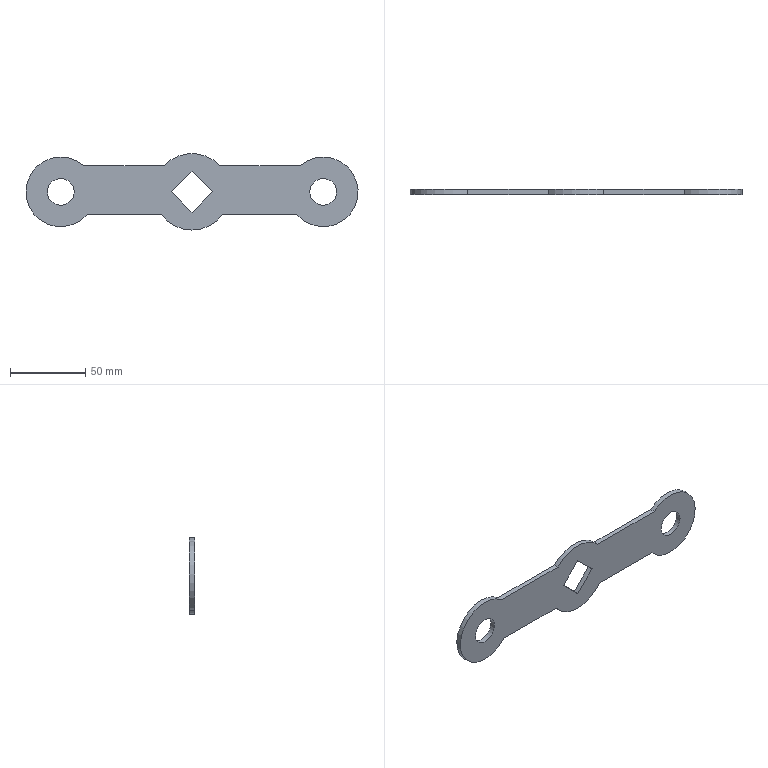Component | NX | ROD | 1 solid | 16 faces | volume 24528 mm3 | plane 10 | cylinder 6 | commonest cylinder face diameters 46.353 x2 50.8 x2 17.78 x2